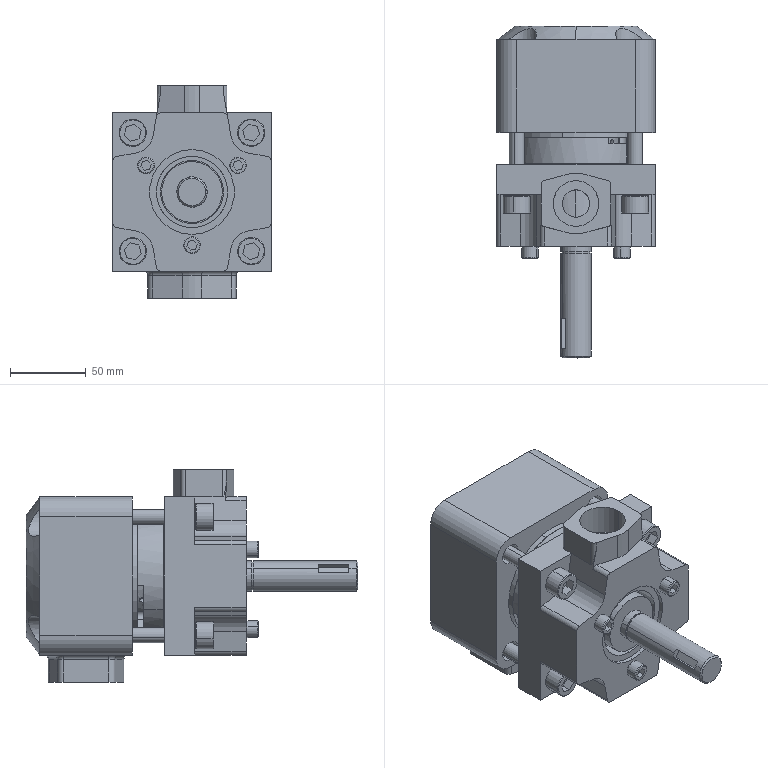Assembly | SolidWorks | mm | 36 component files | 36 solids | 887 faces | box 104 x 218.44 x 140 mm | volume 1084825 mm3 | plane 373 | cylinder 370 | cone 104 | spline 34 | torus 6 | commonest cylinder face diameters 6 x44 3.2 x24 20 x22 18 x16 47 x14 11 x14 26 x13 56 x13
Bill of materials:
10 | 1 |  | Flat annular ring (washer-like) with a central through-hole; moderate axial thickness relative to diameter.
1 | 1 |  | Roughly cubic block with a square flange face that has rounded corners, four corner through-holes, a large internal circular bore/cavity, and a smaller rectangular-section boss projecting from one side.
11 | 1 |  | Thin flat plain ring with a large open center and a narrow radial width.
12 | 1 |  | Thin flat split ring with an open gap at the top and two lugs, one on each side of the gap, each with a small round hole; it resembles an external-type retaining ring.
13 | 1 |  | Thick annular ring/bushing-like disk with a central through-hole whose diameter is roughly 40% of the outer diameter.
14 | 1 |  | Very thin flat split ring with two inward-facing lugs at the gap, each with a small round hole; it resembles an internal-type retaining ring.
15 | 1 |  | Plain thin ring with a narrow radial width and somewhat greater axial width than part-2.
16 | 1 |  | Plain thin ring with a very narrow radial width and a small rectangular cross-section.
17 | 1 |  | Very slender thin ring with a minimal radial and axial width.
19.1 | 1 |  | Long slender cylindrical pin/shaft with an enlarged cylindrical head at one end that has notches/slots in its rim.
19 | 1 |  | Thick annular ring with a central through-hole, very similar in shape to unnamed part.
20 | 4 |  | Cap-screw-like fastener shape: a cylindrical head with a hexagonal socket recess and a long plain cylindrical shank with a chamfered end.
2 | 1 |  | Thin-walled cylindrical ring with four equally spaced small holes in one annular end face.
21 | 3 |  | Headed fastener-like pin: cylindrical head with a hexagonal socket recess and a smaller-diameter plain cylindrical shank.
3 | 12 |  | Flat rectangular plate or block of constant thickness. One edge region appears to be chamfered.
4 | 1 |  | Thick cylindrical disc with twelve radial slots that run axially through the full thickness. Each slot ends in a round hole toward the center. The disc has a central bore with six rectangular keyway-like notches.
5 | 1 |  | Circular disc with a central round bore, two small holes near the rim on opposite sides, and two opposed peripheral notches with angled side walls and curved bottoms.
6 | 1 |  | Stepped turned body with a large flange and smaller coaxial steps, one including a circumferential groove. It has a central bore with a chamfer or counterbore, and two curved arc slots through the flange.
7 | 1 |  | Housing-like block with a large through-bore, a square flange face with four corner through-holes and three smaller countersunk or chamfered holes, and a raised boss on top with its own bore perpendicular to the main bore.
9 | 1 |  | Stepped cylindrical shaft with several diameter sections. It has a rectangular keyway or flat near the larger end, longitudinal slot or spline-like grooves near the step to the smaller end, and narrow circumferential grooves.
Mates:
1. concentric | 1-1 face at (0, 6, 0) dir (0, -1, 0) r 40.5 | 7-1 face at (0, -51.081, 0) dir (0, -1, 0) r 23.5
2. concentric | 1-1 face at (39, 108, 39) dir (0, -1, 0) r 7 | 7-1 face at (39, -40.881, 39) dir (0, 1, 0) r 5.5
3. concentric | 1-1 face at (0, 6, 0) dir (0, -1, 0) r 40.5 | 4-1 face at (0, 40, 0) dir (0, -1, 0) r 28
4. concentric | 1-1 face at (0, 6, 0) dir (0, -1, 0) r 40.5 | 5-1 face at (0, 20, 0) dir (0, -1, 0) r 40
5. concentric | 5-1 face at (0, 20, 0) dir (0, -1, 0) r 40 | 9-1 face at (0, -79.437, 0) dir (0, -1, 0) r 10
6. concentric | 5-1 face at (0, 20, 0) dir (0, -1, 0) r 40 | 6-1 face at (0, -25.3, 0) dir (0, 1, 0) r 40
7. concentric | 2-1 face at (0, 40, 0) dir (0, -1, 0) r 40 | 4-1 face at (0, 40, 0) dir (0, -1, 0) r 28
8. concentric | 19-1 face at (0, 48, 0) dir (0, -1, 0) r 14 | 9-1 face at (0, 22.563, 0) dir (0, -1, 0) r 6
9. concentric | 19.1-1 face at (-36, 8, 0) dir (0, 1, 0) r 1.5 | 5-1 face at (-36, -20, 0) dir (0, 1, 0) r 2.25
10. concentric | 1-1 face at (-36, 48, 0) dir (0, -1, 0) r 3.75 | 19.1-1 face at (-36, 8, 0) dir (0, 1, 0) r 1.5
11. concentric | 10-1 face at (0, -48.332, 0) dir (0, 1, 0) r 20 | 7-1 face at (0, -51.081, 0) dir (0, -1, 0) r 23.5
12. concentric | 16-1 face at (0, 2, 0) dir (0, -1, 0) r 40 | 2-1 face at (0, 40, 0) dir (0, -1, 0) r 40
13. concentric | 15-1 face at (0, -53.3, 0) dir (0, -1, 0) r 20.76 | 6-1 face at (0, -39.3, 0) dir (0, 1, 0) r 23.5
14. concentric | 11-1 face at (0, -30.3, 0) dir (0, -1, 0) r 23.5 | 9-1 face at (0, -79.437, 0) dir (0, -1, 0) r 10
15. concentric | 13-1 face at (0, -39.3, 0) dir (0, -1, 0) r 23.5 | 9-1 face at (0, -79.437, 0) dir (0, -1, 0) r 10
16. concentric | 14-1 edge at (0, -1.8, 0) dir (0, -1, 0) r 21.75 | 4-1 edge at (0, 39, 0) dir (0, 1, 0) r 10
17. concentric | 12-1 edge at (0, -57.937, 0) dir (0, -1, 0) r 9.25 | 9-1 face at (0, -79.437, 0) dir (0, -1, 0) r 10
18. coincident | 12-1 face at (0, -59.437, -0.67) dir (0, -1, 0) | 9-1 face at (0, -59.437, 0) dir (0, 1, 0)
19. coincident | 13-1 face at (0, -53.3, 0) dir (0, -1, 0) | 15-1 face at (0, -53.3, 0) dir (0, 1, 0)
20. coincident | 19-1 edge at (0, 40, 0) dir (0, 1, 0) r 14 | 4-1 face at (0, 40, 0) dir (0, 1, 0)
21. coincident | 1-1 face at (0, 48, 0) dir (0, -1, 0) | 19.1-1 face at (-36, 48, 0) dir (0, -1, 0)
22. coincident | 2-1 face at (0, 20, 0) dir (0, -1, 0) | 4-1 face at (0, 20, 0) dir (0, -1, 0)
23. coincident | 2-1 face at (0, 20, 0) dir (0, -1, 0) | 5-1 face at (0, 20, 0) dir (0, 1, 0)
24. coincident | 16-1 face at (0, 2, 0) dir (0, 1, 0) | 5-1 face at (0, 2, 0) dir (0, -1, 0)
25. coincident | 16-1 face at (0, -3.3, 0) dir (0, -1, 0) | 6-1 face at (0, -3.3, 0) dir (0, 1, 0)
26. concentric | 21-1 face at (30.311, -59.881, 17.5) dir (0, -1, 0) r 3 | 7-1 face at (30.311, -74.881, 17.5) dir (0, -1, 0) r 3.5
27. coincident | 1-1 edge at (0, 48, 0) dir (0, -1, 0) r 14 | 19-1 edge at (0, 48, 0) dir (0, 1, 0) r 14
28. coincident | 21-1 face at (30.311, -74.881, 17.5) dir (0, 1, 0) | 7-1 face at (0, -74.881, 0) dir (0, -1, 0)
29. coincident | 4-1 face at (-4.469, 15, 1.137) dir (0.9691, 0, -0.2466) | 3-12 face at (-10.071, 30.52, -20.874) dir (-0.9691, 0, 0.2466)
30. concentric | 17-1 face at (0, -20.881, 0) dir (0, -1, 0) r 41 | 7-1 face at (0, -23.631, 0) dir (0, 1, 0) r 44.8
31. coincident | 17-1 edge at (0, -23.631, 0) dir (0, 1, 0) r 41 | 7-1 face at (0, -23.631, 0) dir (0, 1, 0)
32. concentric | 19.1-1 face at (-36, 8, 0) dir (0, 1, 0) r 1.5 | 2-1 face at (-36, -70, 0) dir (0, 1, 0) r 2.25
33. coincident | 11-1 face at (0, -30.3, 0) dir (0, 1, 0) | 6-1 face at (0, -30.3, 0) dir (0, -1, 0)
34. concentric | 7-1 face at (39, -40.881, 39) dir (0, 1, 0) r 5.5 | 20-5 face at (39, 48.402, 39) dir (0, -1, 0) r 5